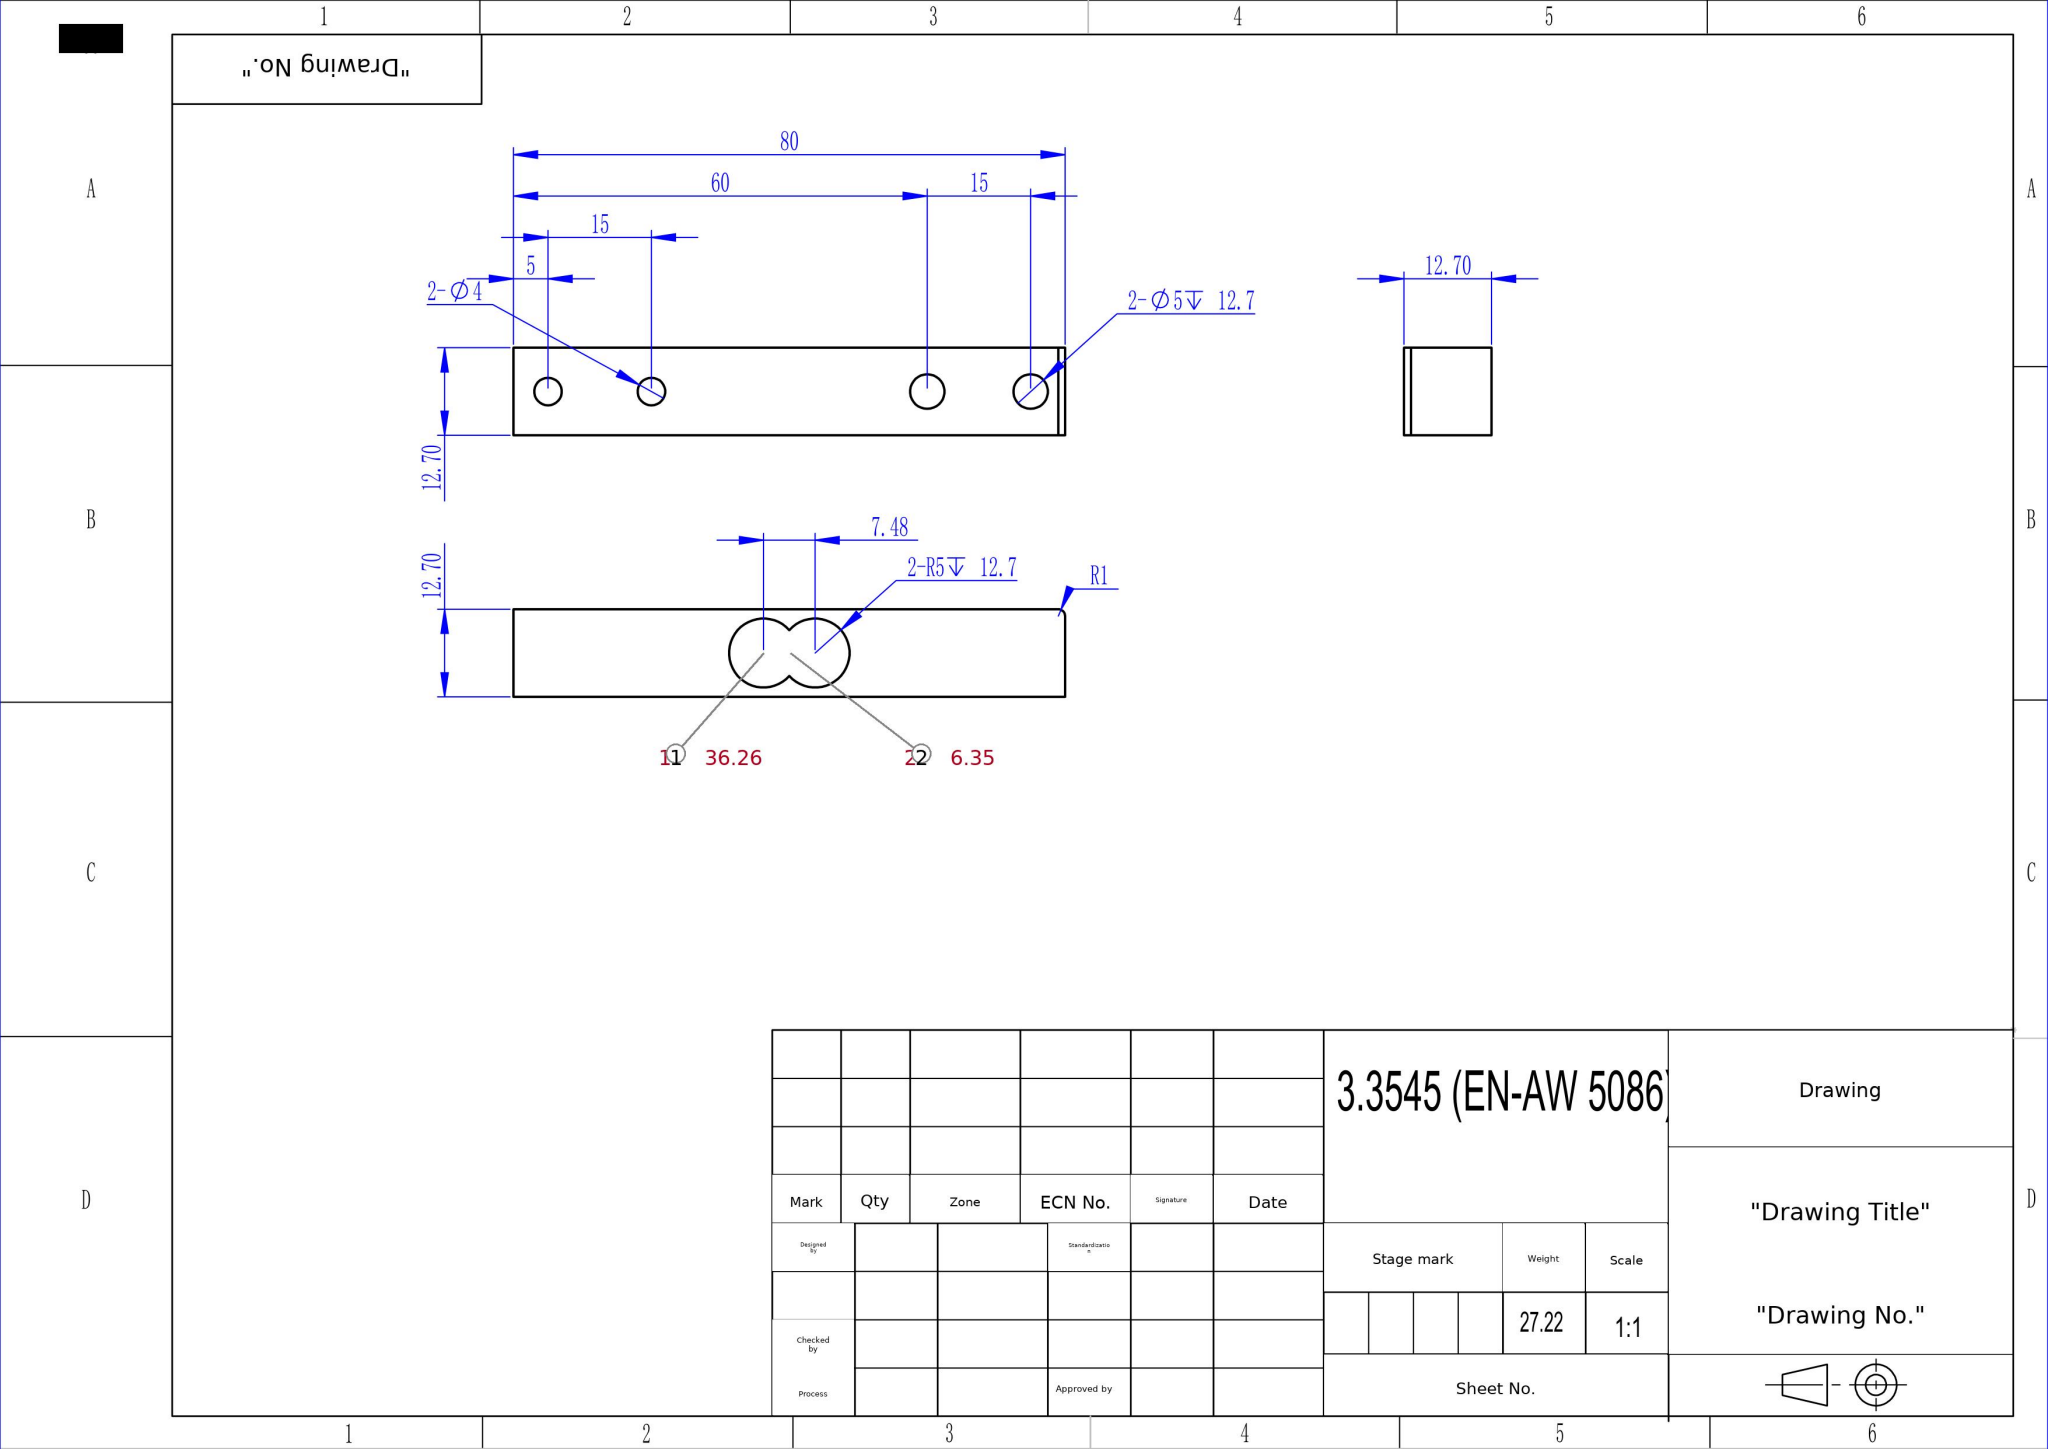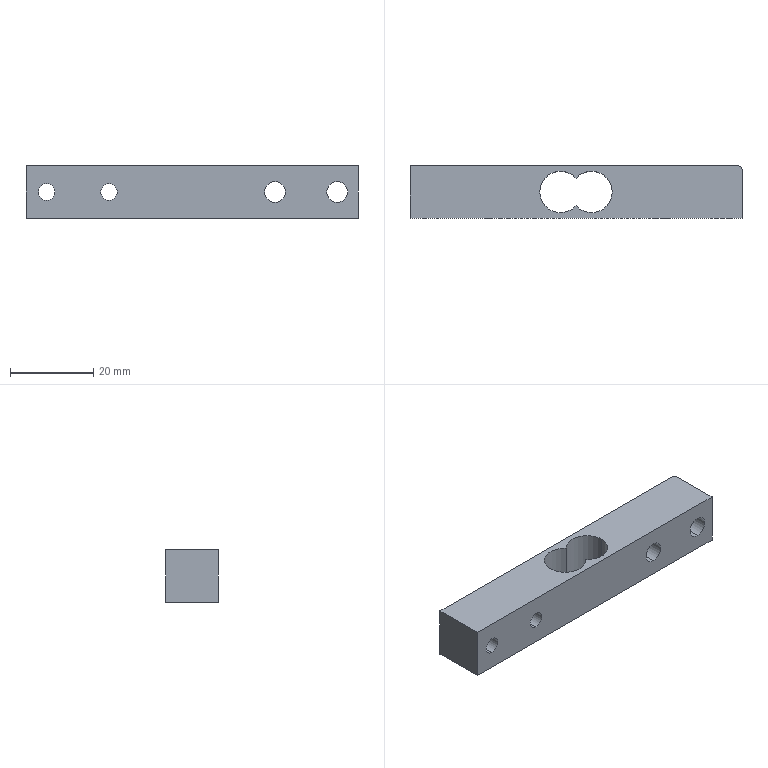Part | SolidWorks | mm | material 3.354 (EN-AW 5086) | 1 solid | 18 faces | box 80 x 12.7 x 12.7 mm | volume 10234 mm3 | cylinder 12 | plane 6 | commonest cylinder face diameters 5 x4 4 x4 10 x3 2 x1
build123d program:
from build123d import *

# Parameters (mm, degrees)
SKETCH1_W           = 80
SKETCH1_H           = 12.7
SKETCH1_R           = 2
BOSS_EXTRUDE1_DEPTH = 12.7
CUT_EXTRUDE1_DEPTH  = 12.7
SKETCH3_R           = 2.5
CUT_EXTRUDE2_DEPTH  = 12.7
FILLET1_R           = 1


with BuildPart() as part:
    # Sketch1 → Boss-Extrude1 (new body)
    with BuildSketch(Plane(origin=(0, 0, 0), x_dir=(1, 0, 0), z_dir=(0, 1, 0))):
        Rectangle(SKETCH1_W, SKETCH1_H)
        with Locations(Location((-35, 0, 0), (0, 0, 270))):
            Circle(SKETCH1_R, mode=Mode.SUBTRACT)
        with Locations(Location((-20, 0, 0), (0, 0, 270))):
            Circle(SKETCH1_R, mode=Mode.SUBTRACT)
        with Locations(Location((20, 0, 0), (0, 0, 90))):
            Circle(SKETCH1_R, mode=Mode.SUBTRACT)
        with Locations(Location((35, 0, 0), (0, 0, 90))):
            Circle(SKETCH1_R, mode=Mode.SUBTRACT)
    extrude(amount=BOSS_EXTRUDE1_DEPTH)

    # Sketch2 → Cut-Extrude1 (cut)
    with BuildSketch(Plane.XY.offset(6.35)):
        with BuildLine():
            ThreePointArc((0, 9.67), (-8.738, 6.35), (0, 3.03))
            ThreePointArc((0, 3.03), (8.738, 6.35), (0, 9.67))
        make_face()
    extrude(amount=-CUT_EXTRUDE1_DEPTH, mode=Mode.SUBTRACT)

    # Sketch3 → Cut-Extrude2 (cut)
    with BuildSketch(Plane(origin=(0, 12.7, 0), x_dir=(1, 0, 0), z_dir=(0, 1, 0))):
        with Locations(Location((20, 0, 0), (0, 0, 270))):
            Circle(SKETCH3_R)
        with Locations(Location((35, 0, 0), (0, 0, 270))):
            Circle(SKETCH3_R)
    extrude(amount=-CUT_EXTRUDE2_DEPTH, mode=Mode.SUBTRACT)

    # Fillet1
    fillet1_edges = [part.edges().sort_by_distance(p)[0] for p in [
        (40, 12.7, 0),
    ]]
    fillet(fillet1_edges, radius=FILLET1_R)


solid = part.part
STEP:
#1=CARTESIAN_POINT('',(20.,0.,-2.5));
#2=VERTEX_POINT('',#1);
#3=CARTESIAN_POINT('',(20.,0.,2.5));
#4=VERTEX_POINT('',#3);
#5=CARTESIAN_POINT('',(20.,0.,0.));
#6=DIRECTION('',(0.,1.,0.));
#7=DIRECTION('',(0.,0.,1.));
#8=AXIS2_PLACEMENT_3D('',#5,#6,#7);
#9=CIRCLE('',#8,2.5);
#10=EDGE_CURVE('',#2,#4,#9,.T.);
#11=ORIENTED_EDGE('',*,*,#10,.F.);
#12=CARTESIAN_POINT('',(20.,12.7,-2.5));
#13=VERTEX_POINT('',#12);
#14=CARTESIAN_POINT('',(20.,0.,-2.5));
#15=DIRECTION('',(0.,1.,0.));
#16=VECTOR('',#15,1000.);
#17=LINE('',#14,#16);
#18=EDGE_CURVE('',#2,#13,#17,.T.);
#19=ORIENTED_EDGE('',*,*,#18,.T.);
#20=CARTESIAN_POINT('',(20.,12.7,2.5));
#21=VERTEX_POINT('',#20);
#22=CARTESIAN_POINT('',(20.,12.7,0.));
#23=DIRECTION('',(0.,1.,0.));
#24=DIRECTION('',(0.,0.,1.));
#25=AXIS2_PLACEMENT_3D('',#22,#23,#24);
#26=CIRCLE('',#25,2.5);
#27=EDGE_CURVE('',#13,#21,#26,.T.);
#28=ORIENTED_EDGE('',*,*,#27,.T.);
#29=CARTESIAN_POINT('',(20.,0.,2.5));
#30=DIRECTION('',(0.,1.,0.));
#31=VECTOR('',#30,1000.);
#32=LINE('',#29,#31);
#33=EDGE_CURVE('',#4,#21,#32,.T.);
#34=ORIENTED_EDGE('',*,*,#33,.F.);
#35=EDGE_LOOP('',(#11,#19,#28,#34));
#36=FACE_OUTER_BOUND('',#35,.T.);
#37=CARTESIAN_POINT('',(20.,0.,0.));
#38=DIRECTION('',(0.,1.,0.));
#39=DIRECTION('',(0.,0.,1.));
#40=AXIS2_PLACEMENT_3D('',#37,#38,#39);
#41=CYLINDRICAL_SURFACE('',#40,2.5);
#42=ADVANCED_FACE('',(#36),#41,.F.);
#43=CARTESIAN_POINT('',(35.,0.,-2.5));
#44=VERTEX_POINT('',#43);
#45=CARTESIAN_POINT('',(35.,0.,2.5));
#46=VERTEX_POINT('',#45);
#47=CARTESIAN_POINT('',(35.,0.,0.));
#48=DIRECTION('',(0.,1.,0.));
#49=DIRECTION('',(0.,0.,1.));
#50=AXIS2_PLACEMENT_3D('',#47,#48,#49);
#51=CIRCLE('',#50,2.5);
#52=EDGE_CURVE('',#44,#46,#51,.T.);
#53=ORIENTED_EDGE('',*,*,#52,.F.);
#54=CARTESIAN_POINT('',(35.,12.7,-2.5));
#55=VERTEX_POINT('',#54);
#56=CARTESIAN_POINT('',(35.,0.,-2.5));
#57=DIRECTION('',(0.,1.,0.));
#58=VECTOR('',#57,1000.);
#59=LINE('',#56,#58);
#60=EDGE_CURVE('',#44,#55,#59,.T.);
#61=ORIENTED_EDGE('',*,*,#60,.T.);
#62=CARTESIAN_POINT('',(35.,12.7,2.5));
#63=VERTEX_POINT('',#62);
#64=CARTESIAN_POINT('',(35.,12.7,0.));
#65=DIRECTION('',(0.,1.,0.));
#66=DIRECTION('',(0.,0.,1.));
#67=AXIS2_PLACEMENT_3D('',#64,#65,#66);
#68=CIRCLE('',#67,2.5);
#69=EDGE_CURVE('',#55,#63,#68,.T.);
#70=ORIENTED_EDGE('',*,*,#69,.T.);
#71=CARTESIAN_POINT('',(35.,0.,2.5));
#72=DIRECTION('',(0.,1.,0.));
#73=VECTOR('',#72,1000.);
#74=LINE('',#71,#73);
#75=EDGE_CURVE('',#46,#63,#74,.T.);
#76=ORIENTED_EDGE('',*,*,#75,.F.);
#77=EDGE_LOOP('',(#53,#61,#70,#76));
#78=FACE_OUTER_BOUND('',#77,.T.);
#79=CARTESIAN_POINT('',(35.,0.,0.));
#80=DIRECTION('',(0.,1.,0.));
#81=DIRECTION('',(0.,0.,1.));
#82=AXIS2_PLACEMENT_3D('',#79,#80,#81);
#83=CYLINDRICAL_SURFACE('',#82,2.5);
#84=ADVANCED_FACE('',(#78),#83,.F.);
#85=CARTESIAN_POINT('',(8.738,6.35,-6.35));
#86=VERTEX_POINT('',#85);
#87=CARTESIAN_POINT('',(-0.,9.67,-6.35));
#88=VERTEX_POINT('',#87);
#89=CARTESIAN_POINT('',(3.738,6.35,-6.35));
#90=DIRECTION('',(0.,0.,1.));
#91=DIRECTION('',(-1.,0.,0.));
#92=AXIS2_PLACEMENT_3D('',#89,#90,#91);
#93=CIRCLE('',#92,5.);
#94=EDGE_CURVE('',#86,#88,#93,.T.);
#95=ORIENTED_EDGE('',*,*,#94,.F.);
#96=CARTESIAN_POINT('',(8.738,6.35,6.35));
#97=VERTEX_POINT('',#96);
#98=CARTESIAN_POINT('',(8.738,6.35,-6.35));
#99=DIRECTION('',(0.,0.,1.));
#100=VECTOR('',#99,1000.);
#101=LINE('',#98,#100);
#102=EDGE_CURVE('',#86,#97,#101,.T.);
#103=ORIENTED_EDGE('',*,*,#102,.T.);
#104=CARTESIAN_POINT('',(-0.,9.67,6.35));
#105=VERTEX_POINT('',#104);
#106=CARTESIAN_POINT('',(3.738,6.35,6.35));
#107=DIRECTION('',(0.,0.,1.));
#108=DIRECTION('',(-1.,0.,0.));
#109=AXIS2_PLACEMENT_3D('',#106,#107,#108);
#110=CIRCLE('',#109,5.);
#111=EDGE_CURVE('',#97,#105,#110,.T.);
#112=ORIENTED_EDGE('',*,*,#111,.T.);
#113=CARTESIAN_POINT('',(-0.,9.67,-6.35));
#114=DIRECTION('',(0.,0.,1.));
#115=VECTOR('',#114,1000.);
#116=LINE('',#113,#115);
#117=EDGE_CURVE('',#88,#105,#116,.T.);
#118=ORIENTED_EDGE('',*,*,#117,.F.);
#119=EDGE_LOOP('',(#95,#103,#112,#118));
#120=FACE_OUTER_BOUND('',#119,.T.);
#121=CARTESIAN_POINT('',(3.738,6.35,-6.35));
#122=DIRECTION('',(0.,0.,1.));
#123=DIRECTION('',(1.,0.,0.));
#124=AXIS2_PLACEMENT_3D('',#121,#122,#123);
#125=CYLINDRICAL_SURFACE('',#124,5.);
#126=ADVANCED_FACE('',(#120),#125,.F.);
#127=CARTESIAN_POINT('',(-20.,12.7,-2.));
#128=VERTEX_POINT('',#127);
#129=CARTESIAN_POINT('',(-20.,12.7,2.));
#130=VERTEX_POINT('',#129);
#131=CARTESIAN_POINT('',(-20.,12.7,0.));
#132=DIRECTION('',(0.,1.,0.));
#133=DIRECTION('',(0.,0.,1.));
#134=AXIS2_PLACEMENT_3D('',#131,#132,#133);
#135=CIRCLE('',#134,2.);
#136=EDGE_CURVE('',#128,#130,#135,.T.);
#137=ORIENTED_EDGE('',*,*,#136,.T.);
#138=CARTESIAN_POINT('',(-20.,0.,2.));
#139=VERTEX_POINT('',#138);
#140=CARTESIAN_POINT('',(-20.,12.7,2.));
#141=DIRECTION('',(0.,-1.,0.));
#142=VECTOR('',#141,1000.);
#143=LINE('',#140,#142);
#144=EDGE_CURVE('',#130,#139,#143,.T.);
#145=ORIENTED_EDGE('',*,*,#144,.T.);
#146=CARTESIAN_POINT('',(-20.,0.,-2.));
#147=VERTEX_POINT('',#146);
#148=CARTESIAN_POINT('',(-20.,0.,0.));
#149=DIRECTION('',(0.,1.,0.));
#150=DIRECTION('',(0.,0.,1.));
#151=AXIS2_PLACEMENT_3D('',#148,#149,#150);
#152=CIRCLE('',#151,2.);
#153=EDGE_CURVE('',#147,#139,#152,.T.);
#154=ORIENTED_EDGE('',*,*,#153,.F.);
#155=CARTESIAN_POINT('',(-20.,12.7,-2.));
#156=DIRECTION('',(0.,-1.,0.));
#157=VECTOR('',#156,1000.);
#158=LINE('',#155,#157);
#159=EDGE_CURVE('',#128,#147,#158,.T.);
#160=ORIENTED_EDGE('',*,*,#159,.F.);
#161=EDGE_LOOP('',(#137,#145,#154,#160));
#162=FACE_OUTER_BOUND('',#161,.T.);
#163=CARTESIAN_POINT('',(-20.,12.7,0.));
#164=DIRECTION('',(0.,-1.,0.));
#165=DIRECTION('',(0.,0.,-1.));
#166=AXIS2_PLACEMENT_3D('',#163,#164,#165);
#167=CYLINDRICAL_SURFACE('',#166,2.);
#168=ADVANCED_FACE('',(#162),#167,.F.);
#169=CARTESIAN_POINT('',(-35.,12.7,-2.));
#170=VERTEX_POINT('',#169);
#171=CARTESIAN_POINT('',(-35.,12.7,2.));
#172=VERTEX_POINT('',#171);
#173=CARTESIAN_POINT('',(-35.,12.7,0.));
#174=DIRECTION('',(0.,1.,0.));
#175=DIRECTION('',(0.,0.,1.));
#176=AXIS2_PLACEMENT_3D('',#173,#174,#175);
#177=CIRCLE('',#176,2.);
#178=EDGE_CURVE('',#170,#172,#177,.T.);
#179=ORIENTED_EDGE('',*,*,#178,.T.);
#180=CARTESIAN_POINT('',(-35.,0.,2.));
#181=VERTEX_POINT('',#180);
#182=CARTESIAN_POINT('',(-35.,12.7,2.));
#183=DIRECTION('',(0.,-1.,0.));
#184=VECTOR('',#183,1000.);
#185=LINE('',#182,#184);
#186=EDGE_CURVE('',#172,#181,#185,.T.);
#187=ORIENTED_EDGE('',*,*,#186,.T.);
#188=CARTESIAN_POINT('',(-35.,0.,-2.));
#189=VERTEX_POINT('',#188);
#190=CARTESIAN_POINT('',(-35.,0.,0.));
#191=DIRECTION('',(0.,1.,0.));
#192=DIRECTION('',(0.,0.,1.));
#193=AXIS2_PLACEMENT_3D('',#190,#191,#192);
#194=CIRCLE('',#193,2.);
#195=EDGE_CURVE('',#189,#181,#194,.T.);
#196=ORIENTED_EDGE('',*,*,#195,.F.);
#197=CARTESIAN_POINT('',(-35.,12.7,-2.));
#198=DIRECTION('',(0.,-1.,0.));
#199=VECTOR('',#198,1000.);
#200=LINE('',#197,#199);
#201=EDGE_CURVE('',#170,#189,#200,.T.);
#202=ORIENTED_EDGE('',*,*,#201,.F.);
#203=EDGE_LOOP('',(#179,#187,#196,#202));
#204=FACE_OUTER_BOUND('',#203,.T.);
#205=CARTESIAN_POINT('',(-35.,12.7,0.));
#206=DIRECTION('',(0.,-1.,0.));
#207=DIRECTION('',(0.,0.,-1.));
#208=AXIS2_PLACEMENT_3D('',#205,#206,#207);
#209=CYLINDRICAL_SURFACE('',#208,2.);
#210=ADVANCED_FACE('',(#204),#209,.F.);
#211=CARTESIAN_POINT('',(20.,12.7,0.));
#212=DIRECTION('',(0.,1.,0.));
#213=DIRECTION('',(0.,0.,1.));
#214=AXIS2_PLACEMENT_3D('',#211,#212,#213);
#215=CIRCLE('',#214,2.5);
#216=EDGE_CURVE('',#21,#13,#215,.T.);
#217=ORIENTED_EDGE('',*,*,#216,.F.);
#218=ORIENTED_EDGE('',*,*,#27,.F.);
#219=EDGE_LOOP('',(#217,#218));
#220=FACE_BOUND('',#219,.T.);
#221=CARTESIAN_POINT('',(35.,12.7,0.));
#222=DIRECTION('',(0.,1.,0.));
#223=DIRECTION('',(0.,0.,1.));
#224=AXIS2_PLACEMENT_3D('',#221,#222,#223);
#225=CIRCLE('',#224,2.5);
#226=EDGE_CURVE('',#63,#55,#225,.T.);
#227=ORIENTED_EDGE('',*,*,#226,.F.);
#228=ORIENTED_EDGE('',*,*,#69,.F.);
#229=EDGE_LOOP('',(#227,#228));
#230=FACE_BOUND('',#229,.T.);
#231=ORIENTED_EDGE('',*,*,#178,.F.);
#232=CARTESIAN_POINT('',(-35.,12.7,0.));
#233=DIRECTION('',(0.,1.,0.));
#234=DIRECTION('',(0.,0.,1.));
#235=AXIS2_PLACEMENT_3D('',#232,#233,#234);
#236=CIRCLE('',#235,2.);
#237=EDGE_CURVE('',#172,#170,#236,.T.);
#238=ORIENTED_EDGE('',*,*,#237,.F.);
#239=EDGE_LOOP('',(#231,#238));
#240=FACE_BOUND('',#239,.T.);
#241=CARTESIAN_POINT('',(-40.,12.7,6.35));
#242=VERTEX_POINT('',#241);
#243=CARTESIAN_POINT('',(39.,12.7,6.35));
#244=VERTEX_POINT('',#243);
#245=CARTESIAN_POINT('',(-40.,12.7,6.35));
#246=DIRECTION('',(1.,0.,0.));
#247=VECTOR('',#246,1000.);
#248=LINE('',#245,#247);
#249=EDGE_CURVE('',#242,#244,#248,.T.);
#250=ORIENTED_EDGE('',*,*,#249,.T.);
#251=CARTESIAN_POINT('',(39.,12.7,-6.35));
#252=VERTEX_POINT('',#251);
#253=CARTESIAN_POINT('',(39.,12.7,-6.35));
#254=DIRECTION('',(0.,0.,-1.));
#255=VECTOR('',#254,1000.);
#256=LINE('',#253,#255);
#257=EDGE_CURVE('',#244,#252,#256,.T.);
#258=ORIENTED_EDGE('',*,*,#257,.T.);
#259=CARTESIAN_POINT('',(-40.,12.7,-6.35));
#260=VERTEX_POINT('',#259);
#261=CARTESIAN_POINT('',(-40.,12.7,-6.35));
#262=DIRECTION('',(-1.,0.,0.));
#263=VECTOR('',#262,1000.);
#264=LINE('',#261,#263);
#265=EDGE_CURVE('',#252,#260,#264,.T.);
#266=ORIENTED_EDGE('',*,*,#265,.T.);
#267=CARTESIAN_POINT('',(-40.,12.7,-6.35));
#268=DIRECTION('',(0.,0.,1.));
#269=VECTOR('',#268,1000.);
#270=LINE('',#267,#269);
#271=EDGE_CURVE('',#260,#242,#270,.T.);
#272=ORIENTED_EDGE('',*,*,#271,.T.);
#273=EDGE_LOOP('',(#250,#258,#266,#272));
#274=FACE_OUTER_BOUND('',#273,.T.);
#275=ORIENTED_EDGE('',*,*,#136,.F.);
#276=CARTESIAN_POINT('',(-20.,12.7,0.));
#277=DIRECTION('',(0.,1.,0.));
#278=DIRECTION('',(0.,0.,1.));
#279=AXIS2_PLACEMENT_3D('',#276,#277,#278);
#280=CIRCLE('',#279,2.);
#281=EDGE_CURVE('',#130,#128,#280,.T.);
#282=ORIENTED_EDGE('',*,*,#281,.F.);
#283=EDGE_LOOP('',(#275,#282));
#284=FACE_BOUND('',#283,.T.);
#285=CARTESIAN_POINT('',(0.,12.7,0.));
#286=DIRECTION('',(0.,1.,0.));
#287=DIRECTION('',(0.,0.,1.));
#288=AXIS2_PLACEMENT_3D('',#285,#286,#287);
#289=PLANE('',#288);
#290=ADVANCED_FACE('',(#220,#230,#240,#274,#284),#289,.T.);
#291=CARTESIAN_POINT('',(20.,0.,0.));
#292=DIRECTION('',(0.,1.,0.));
#293=DIRECTION('',(0.,0.,1.));
#294=AXIS2_PLACEMENT_3D('',#291,#292,#293);
#295=CIRCLE('',#294,2.5);
#296=EDGE_CURVE('',#4,#2,#295,.T.);
#297=ORIENTED_EDGE('',*,*,#296,.T.);
#298=ORIENTED_EDGE('',*,*,#10,.T.);
#299=EDGE_LOOP('',(#297,#298));
#300=FACE_BOUND('',#299,.T.);
#301=CARTESIAN_POINT('',(35.,0.,0.));
#302=DIRECTION('',(0.,1.,0.));
#303=DIRECTION('',(0.,0.,1.));
#304=AXIS2_PLACEMENT_3D('',#301,#302,#303);
#305=CIRCLE('',#304,2.5);
#306=EDGE_CURVE('',#46,#44,#305,.T.);
#307=ORIENTED_EDGE('',*,*,#306,.T.);
#308=ORIENTED_EDGE('',*,*,#52,.T.);
#309=EDGE_LOOP('',(#307,#308));
#310=FACE_BOUND('',#309,.T.);
#311=CARTESIAN_POINT('',(40.,0.,6.35));
#312=VERTEX_POINT('',#311);
#313=CARTESIAN_POINT('',(40.,0.,-6.35));
#314=VERTEX_POINT('',#313);
#315=CARTESIAN_POINT('',(40.,0.,-6.35));
#316=DIRECTION('',(0.,0.,-1.));
#317=VECTOR('',#316,1000.);
#318=LINE('',#315,#317);
#319=EDGE_CURVE('',#312,#314,#318,.T.);
#320=ORIENTED_EDGE('',*,*,#319,.F.);
#321=CARTESIAN_POINT('',(-40.,0.,6.35));
#322=VERTEX_POINT('',#321);
#323=CARTESIAN_POINT('',(-40.,0.,6.35));
#324=DIRECTION('',(1.,0.,0.));
#325=VECTOR('',#324,1000.);
#326=LINE('',#323,#325);
#327=EDGE_CURVE('',#322,#312,#326,.T.);
#328=ORIENTED_EDGE('',*,*,#327,.F.);
#329=CARTESIAN_POINT('',(-40.,0.,-6.35));
#330=VERTEX_POINT('',#329);
#331=CARTESIAN_POINT('',(-40.,0.,-6.35));
#332=DIRECTION('',(0.,0.,1.));
#333=VECTOR('',#332,1000.);
#334=LINE('',#331,#333);
#335=EDGE_CURVE('',#330,#322,#334,.T.);
#336=ORIENTED_EDGE('',*,*,#335,.F.);
#337=CARTESIAN_POINT('',(-40.,0.,-6.35));
#338=DIRECTION('',(-1.,0.,0.));
#339=VECTOR('',#338,1000.);
#340=LINE('',#337,#339);
#341=EDGE_CURVE('',#314,#330,#340,.T.);
#342=ORIENTED_EDGE('',*,*,#341,.F.);
#343=EDGE_LOOP('',(#320,#328,#336,#342));
#344=FACE_OUTER_BOUND('',#343,.T.);
#345=ORIENTED_EDGE('',*,*,#195,.T.);
#346=CARTESIAN_POINT('',(-35.,0.,0.));
#347=DIRECTION('',(0.,1.,0.));
#348=DIRECTION('',(0.,0.,1.));
#349=AXIS2_PLACEMENT_3D('',#346,#347,#348);
#350=CIRCLE('',#349,2.);
#351=EDGE_CURVE('',#181,#189,#350,.T.);
#352=ORIENTED_EDGE('',*,*,#351,.T.);
#353=EDGE_LOOP('',(#345,#352));
#354=FACE_BOUND('',#353,.T.);
#355=ORIENTED_EDGE('',*,*,#153,.T.);
#356=CARTESIAN_POINT('',(-20.,0.,0.));
#357=DIRECTION('',(0.,1.,0.));
#358=DIRECTION('',(0.,0.,1.));
#359=AXIS2_PLACEMENT_3D('',#356,#357,#358);
#360=CIRCLE('',#359,2.);
#361=EDGE_CURVE('',#139,#147,#360,.T.);
#362=ORIENTED_EDGE('',*,*,#361,.T.);
#363=EDGE_LOOP('',(#355,#362));
#364=FACE_BOUND('',#363,.T.);
#365=CARTESIAN_POINT('',(0.,0.,0.));
#366=DIRECTION('',(0.,1.,0.));
#367=DIRECTION('',(0.,0.,1.));
#368=AXIS2_PLACEMENT_3D('',#365,#366,#367);
#369=PLANE('',#368);
#370=ADVANCED_FACE('',(#300,#310,#344,#354,#364),#369,.F.);
#371=CARTESIAN_POINT('',(40.,11.7,-6.35));
#372=VERTEX_POINT('',#371);
#373=CARTESIAN_POINT('',(40.,12.7,-6.35));
#374=DIRECTION('',(0.,-1.,0.));
#375=VECTOR('',#374,1000.);
#376=LINE('',#373,#375);
#377=EDGE_CURVE('',#372,#314,#376,.T.);
#378=ORIENTED_EDGE('',*,*,#377,.F.);
#379=CARTESIAN_POINT('',(40.,11.7,6.35));
#380=VERTEX_POINT('',#379);
#381=CARTESIAN_POINT('',(40.,11.7,6.35));
#382=DIRECTION('',(0.,0.,1.));
#383=VECTOR('',#382,1000.);
#384=LINE('',#381,#383);
#385=EDGE_CURVE('',#372,#380,#384,.T.);
#386=ORIENTED_EDGE('',*,*,#385,.T.);
#387=CARTESIAN_POINT('',(40.,12.7,6.35));
#388=DIRECTION('',(0.,-1.,0.));
#389=VECTOR('',#388,1000.);
#390=LINE('',#387,#389);
#391=EDGE_CURVE('',#380,#312,#390,.T.);
#392=ORIENTED_EDGE('',*,*,#391,.T.);
#393=ORIENTED_EDGE('',*,*,#319,.T.);
#394=EDGE_LOOP('',(#378,#386,#392,#393));
#395=FACE_OUTER_BOUND('',#394,.T.);
#396=CARTESIAN_POINT('',(40.,12.7,-6.35));
#397=DIRECTION('',(-1.,0.,0.));
#398=DIRECTION('',(0.,0.,1.));
#399=AXIS2_PLACEMENT_3D('',#396,#397,#398);
#400=PLANE('',#399);
#401=ADVANCED_FACE('',(#395),#400,.F.);
#402=CARTESIAN_POINT('',(-0.,3.03,-6.35));
#403=VERTEX_POINT('',#402);
#404=CARTESIAN_POINT('',(-3.738,6.35,-6.35));
#405=DIRECTION('',(0.,0.,1.));
#406=DIRECTION('',(1.,0.,0.));
#407=AXIS2_PLACEMENT_3D('',#404,#405,#406);
#408=CIRCLE('',#407,5.);
#409=EDGE_CURVE('',#88,#403,#408,.T.);
#410=ORIENTED_EDGE('',*,*,#409,.T.);
#411=CARTESIAN_POINT('',(3.738,6.35,-6.35));
#412=DIRECTION('',(0.,0.,1.));
#413=DIRECTION('',(-1.,0.,0.));
#414=AXIS2_PLACEMENT_3D('',#411,#412,#413);
#415=CIRCLE('',#414,5.);
#416=EDGE_CURVE('',#403,#86,#415,.T.);
#417=ORIENTED_EDGE('',*,*,#416,.T.);
#418=ORIENTED_EDGE('',*,*,#94,.T.);
#419=EDGE_LOOP('',(#410,#417,#418));
#420=FACE_BOUND('',#419,.T.);
#421=ORIENTED_EDGE('',*,*,#265,.F.);
#422=CARTESIAN_POINT('',(39.,11.7,-6.35));
#423=DIRECTION('',(0.,0.,-1.));
#424=DIRECTION('',(1.,0.,0.));
#425=AXIS2_PLACEMENT_3D('',#422,#423,#424);
#426=CIRCLE('',#425,1.);
#427=EDGE_CURVE('',#252,#372,#426,.T.);
#428=ORIENTED_EDGE('',*,*,#427,.T.);
#429=ORIENTED_EDGE('',*,*,#377,.T.);
#430=ORIENTED_EDGE('',*,*,#341,.T.);
#431=CARTESIAN_POINT('',(-40.,12.7,-6.35));
#432=DIRECTION('',(0.,-1.,0.));
#433=VECTOR('',#432,1000.);
#434=LINE('',#431,#433);
#435=EDGE_CURVE('',#260,#330,#434,.T.);
#436=ORIENTED_EDGE('',*,*,#435,.F.);
#437=EDGE_LOOP('',(#421,#428,#429,#430,#436));
#438=FACE_OUTER_BOUND('',#437,.T.);
#439=CARTESIAN_POINT('',(-40.,12.7,-6.35));
#440=DIRECTION('',(0.,0.,1.));
#441=DIRECTION('',(1.,0.,0.));
#442=AXIS2_PLACEMENT_3D('',#439,#440,#441);
#443=PLANE('',#442);
#444=ADVANCED_FACE('',(#420,#438),#443,.F.);
#445=ORIENTED_EDGE('',*,*,#335,.T.);
#446=CARTESIAN_POINT('',(-40.,12.7,6.35));
#447=DIRECTION('',(0.,-1.,0.));
#448=VECTOR('',#447,1000.);
#449=LINE('',#446,#448);
#450=EDGE_CURVE('',#242,#322,#449,.T.);
#451=ORIENTED_EDGE('',*,*,#450,.F.);
#452=ORIENTED_EDGE('',*,*,#271,.F.);
#453=ORIENTED_EDGE('',*,*,#435,.T.);
#454=EDGE_LOOP('',(#445,#451,#452,#453));
#455=FACE_OUTER_BOUND('',#454,.T.);
#456=CARTESIAN_POINT('',(-40.,12.7,-6.35));
#457=DIRECTION('',(1.,0.,0.));
#458=DIRECTION('',(0.,0.,-1.));
#459=AXIS2_PLACEMENT_3D('',#456,#457,#458);
#460=PLANE('',#459);
#461=ADVANCED_FACE('',(#455),#460,.F.);
#462=CARTESIAN_POINT('',(-0.,3.03,6.35));
#463=VERTEX_POINT('',#462);
#464=CARTESIAN_POINT('',(-3.738,6.35,6.35));
#465=DIRECTION('',(0.,0.,1.));
#466=DIRECTION('',(1.,0.,0.));
#467=AXIS2_PLACEMENT_3D('',#464,#465,#466);
#468=CIRCLE('',#467,5.);
#469=EDGE_CURVE('',#105,#463,#468,.T.);
#470=ORIENTED_EDGE('',*,*,#469,.F.);
#471=ORIENTED_EDGE('',*,*,#111,.F.);
#472=CARTESIAN_POINT('',(3.738,6.35,6.35));
#473=DIRECTION('',(0.,0.,1.));
#474=DIRECTION('',(-1.,0.,0.));
#475=AXIS2_PLACEMENT_3D('',#472,#473,#474);
#476=CIRCLE('',#475,5.);
#477=EDGE_CURVE('',#463,#97,#476,.T.);
#478=ORIENTED_EDGE('',*,*,#477,.F.);
#479=EDGE_LOOP('',(#470,#471,#478));
#480=FACE_BOUND('',#479,.T.);
#481=ORIENTED_EDGE('',*,*,#391,.F.);
#482=CARTESIAN_POINT('',(39.,11.7,6.35));
#483=DIRECTION('',(0.,0.,1.));
#484=DIRECTION('',(-1.,0.,0.));
#485=AXIS2_PLACEMENT_3D('',#482,#483,#484);
#486=CIRCLE('',#485,1.);
#487=EDGE_CURVE('',#380,#244,#486,.T.);
#488=ORIENTED_EDGE('',*,*,#487,.T.);
#489=ORIENTED_EDGE('',*,*,#249,.F.);
#490=ORIENTED_EDGE('',*,*,#450,.T.);
#491=ORIENTED_EDGE('',*,*,#327,.T.);
#492=EDGE_LOOP('',(#481,#488,#489,#490,#491));
#493=FACE_OUTER_BOUND('',#492,.T.);
#494=CARTESIAN_POINT('',(-40.,12.7,6.35));
#495=DIRECTION('',(0.,0.,-1.));
#496=DIRECTION('',(-1.,0.,0.));
#497=AXIS2_PLACEMENT_3D('',#494,#495,#496);
#498=PLANE('',#497);
#499=ADVANCED_FACE('',(#480,#493),#498,.F.);
#500=ORIENTED_EDGE('',*,*,#186,.F.);
#501=ORIENTED_EDGE('',*,*,#237,.T.);
#502=ORIENTED_EDGE('',*,*,#201,.T.);
#503=ORIENTED_EDGE('',*,*,#351,.F.);
#504=EDGE_LOOP('',(#500,#501,#502,#503));
#505=FACE_OUTER_BOUND('',#504,.T.);
#506=CARTESIAN_POINT('',(-35.,12.7,0.));
#507=DIRECTION('',(0.,-1.,0.));
#508=DIRECTION('',(0.,0.,-1.));
#509=AXIS2_PLACEMENT_3D('',#506,#507,#508);
#510=CYLINDRICAL_SURFACE('',#509,2.);
#511=ADVANCED_FACE('',(#505),#510,.F.);
#512=ORIENTED_EDGE('',*,*,#144,.F.);
#513=ORIENTED_EDGE('',*,*,#281,.T.);
#514=ORIENTED_EDGE('',*,*,#159,.T.);
#515=ORIENTED_EDGE('',*,*,#361,.F.);
#516=EDGE_LOOP('',(#512,#513,#514,#515));
#517=FACE_OUTER_BOUND('',#516,.T.);
#518=CARTESIAN_POINT('',(-20.,12.7,0.));
#519=DIRECTION('',(0.,-1.,0.));
#520=DIRECTION('',(0.,0.,-1.));
#521=AXIS2_PLACEMENT_3D('',#518,#519,#520);
#522=CYLINDRICAL_SURFACE('',#521,2.);
#523=ADVANCED_FACE('',(#517),#522,.F.);
#524=ORIENTED_EDGE('',*,*,#102,.F.);
#525=ORIENTED_EDGE('',*,*,#416,.F.);
#526=CARTESIAN_POINT('',(-0.,3.03,-6.35));
#527=DIRECTION('',(0.,0.,1.));
#528=VECTOR('',#527,1000.);
#529=LINE('',#526,#528);
#530=EDGE_CURVE('',#403,#463,#529,.T.);
#531=ORIENTED_EDGE('',*,*,#530,.T.);
#532=ORIENTED_EDGE('',*,*,#477,.T.);
#533=EDGE_LOOP('',(#524,#525,#531,#532));
#534=FACE_OUTER_BOUND('',#533,.T.);
#535=CARTESIAN_POINT('',(3.738,6.35,-6.35));
#536=DIRECTION('',(0.,0.,1.));
#537=DIRECTION('',(1.,0.,0.));
#538=AXIS2_PLACEMENT_3D('',#535,#536,#537);
#539=CYLINDRICAL_SURFACE('',#538,5.);
#540=ADVANCED_FACE('',(#534),#539,.F.);
#541=ORIENTED_EDGE('',*,*,#469,.T.);
#542=ORIENTED_EDGE('',*,*,#530,.F.);
#543=ORIENTED_EDGE('',*,*,#409,.F.);
#544=ORIENTED_EDGE('',*,*,#117,.T.);
#545=EDGE_LOOP('',(#541,#542,#543,#544));
#546=FACE_OUTER_BOUND('',#545,.T.);
#547=CARTESIAN_POINT('',(-3.738,6.35,-6.35));
#548=DIRECTION('',(0.,0.,1.));
#549=DIRECTION('',(1.,0.,0.));
#550=AXIS2_PLACEMENT_3D('',#547,#548,#549);
#551=CYLINDRICAL_SURFACE('',#550,5.);
#552=ADVANCED_FACE('',(#546),#551,.F.);
#553=ORIENTED_EDGE('',*,*,#60,.F.);
#554=ORIENTED_EDGE('',*,*,#306,.F.);
#555=ORIENTED_EDGE('',*,*,#75,.T.);
#556=ORIENTED_EDGE('',*,*,#226,.T.);
#557=EDGE_LOOP('',(#553,#554,#555,#556));
#558=FACE_OUTER_BOUND('',#557,.T.);
#559=CARTESIAN_POINT('',(35.,0.,0.));
#560=DIRECTION('',(0.,1.,0.));
#561=DIRECTION('',(0.,0.,1.));
#562=AXIS2_PLACEMENT_3D('',#559,#560,#561);
#563=CYLINDRICAL_SURFACE('',#562,2.5);
#564=ADVANCED_FACE('',(#558),#563,.F.);
#565=ORIENTED_EDGE('',*,*,#18,.F.);
#566=ORIENTED_EDGE('',*,*,#296,.F.);
#567=ORIENTED_EDGE('',*,*,#33,.T.);
#568=ORIENTED_EDGE('',*,*,#216,.T.);
#569=EDGE_LOOP('',(#565,#566,#567,#568));
#570=FACE_OUTER_BOUND('',#569,.T.);
#571=CARTESIAN_POINT('',(20.,0.,0.));
#572=DIRECTION('',(0.,1.,0.));
#573=DIRECTION('',(0.,0.,1.));
#574=AXIS2_PLACEMENT_3D('',#571,#572,#573);
#575=CYLINDRICAL_SURFACE('',#574,2.5);
#576=ADVANCED_FACE('',(#570),#575,.F.);
#577=ORIENTED_EDGE('',*,*,#487,.F.);
#578=ORIENTED_EDGE('',*,*,#385,.F.);
#579=ORIENTED_EDGE('',*,*,#427,.F.);
#580=ORIENTED_EDGE('',*,*,#257,.F.);
#581=EDGE_LOOP('',(#577,#578,#579,#580));
#582=FACE_OUTER_BOUND('',#581,.T.);
#583=CARTESIAN_POINT('',(39.,11.7,0.));
#584=DIRECTION('',(0.,0.,1.));
#585=DIRECTION('',(1.,0.,0.));
#586=AXIS2_PLACEMENT_3D('',#583,#584,#585);
#587=CYLINDRICAL_SURFACE('',#586,1.);
#588=ADVANCED_FACE('',(#582),#587,.T.);
#589=CLOSED_SHELL('',(#42,#84,#126,#168,#210,#290,#370,#401,#444,#461,#499,#511,#523,#540,#552,#564,#576,#588));
#590=MANIFOLD_SOLID_BREP('',#589);
#591=CARTESIAN_POINT('',(0.,0.,0.));
#592=DIRECTION('',(0.,0.,1.));
#593=DIRECTION('',(1.,0.,0.));
#594=AXIS2_PLACEMENT_3D('',#591,#592,#593);
#595=(LENGTH_UNIT()NAMED_UNIT(*)SI_UNIT(.MILLI.,.METRE.));
#596=UNCERTAINTY_MEASURE_WITH_UNIT(LENGTH_MEASURE(0.00001),#595,'','');
#597=(NAMED_UNIT(*)PLANE_ANGLE_UNIT()SI_UNIT($,.RADIAN.));
#598=(NAMED_UNIT(*)SI_UNIT($,.STERADIAN.)SOLID_ANGLE_UNIT());
#599=(GEOMETRIC_REPRESENTATION_CONTEXT(3)GLOBAL_UNCERTAINTY_ASSIGNED_CONTEXT((#596))GLOBAL_UNIT_ASSIGNED_CONTEXT((#595,#597,#598))REPRESENTATION_CONTEXT('',''));
#600=ADVANCED_BREP_SHAPE_REPRESENTATION('',(#590,#594),#599);